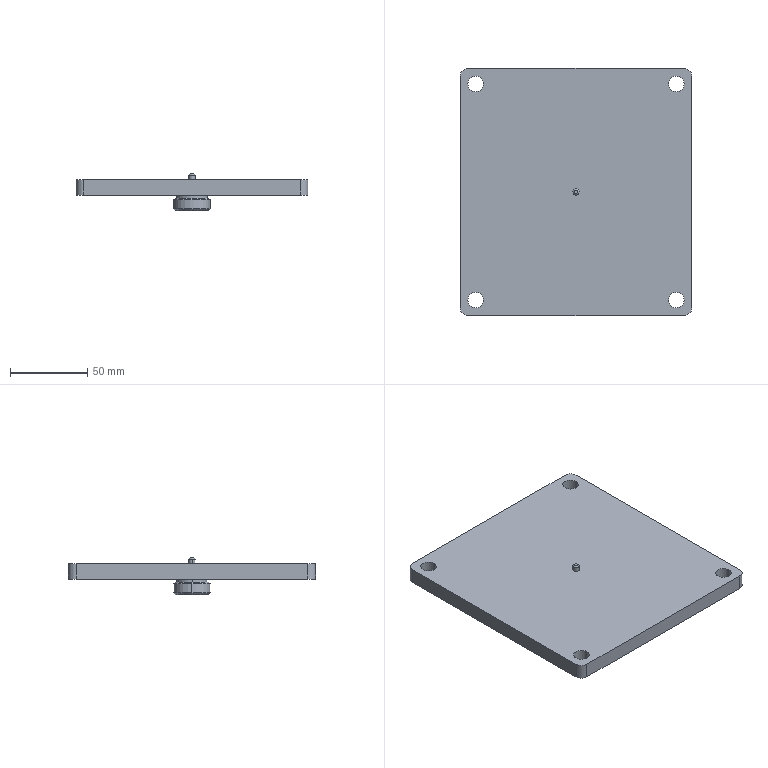Component | SolidWorks | GearboxTopCover-1 | 1 solid | 33 faces | box 150 x 160 x 24 mm | volume 240863 mm3 | cylinder 18 | plane 9 | cone 6 | commonest cylinder face diameters 10 x12 24 x2 4 x2 20 x2
build123d program:
from build123d import *

# Parameters (mm, degrees)
SKETCH1_4_W         = 160
SKETCH1_4_H         = 150
SKETCH1_4_R         = 10
SKETCH1_4_R_2       = 5
BOSS_EXTRUDE1_DEPTH = 10
FILLET1_R           = 5
SKETCH1_3_R         = 10
SKETCH1_3_R_2       = 2
BOSS_EXTRUDE2_DEPTH = 12
SKETCH1_4_2_R       = 2
BOSS_EXTRUDE3_DEPTH = 4
CHAMFER1_SIZE       = 1
SKETCH4_R           = 12
BOSS_EXTRUDE4_DEPTH = 8
CHAMFER2_SIZE       = 1


with BuildPart() as part:
    # Sketch1_4 → Boss-Extrude1 (new body)
    with BuildSketch(Plane(origin=(0, 0, 0), x_dir=(1, 0, 0), z_dir=(0, 1, 0))):
        Rectangle(SKETCH1_4_W, SKETCH1_4_H)
        with Locations(Location((0, 0, 0), (0, 0, 270))):
            Circle(SKETCH1_4_R, mode=Mode.SUBTRACT)
        with Locations(Location((-70, -65, 0), (0, 0, 270))):
            Circle(SKETCH1_4_R_2, mode=Mode.SUBTRACT)
        with Locations(Location((-70, 65, 0), (0, 0, 270))):
            Circle(SKETCH1_4_R_2, mode=Mode.SUBTRACT)
        with Locations(Location((70, -65, 0), (0, 0, 270))):
            Circle(SKETCH1_4_R_2, mode=Mode.SUBTRACT)
        with Locations(Location((70, 65, 0), (0, 0, 270))):
            Circle(SKETCH1_4_R_2, mode=Mode.SUBTRACT)
    extrude(amount=BOSS_EXTRUDE1_DEPTH)

    # Fillet1
    fillet1_edges = [part.edges().sort_by_distance(p)[0] for p in [
        (-80, 5, 75),
        (-80, 5, -75),
        (80, 5, -75),
        (80, 5, 75),
    ]]
    fillet(fillet1_edges, radius=FILLET1_R)

    # Sketch1_3 → Boss-Extrude2 (add)
    # profile 1 of 2: a face of its own
    with BuildSketch(Plane(origin=(0, 0, 0), x_dir=(1, 0, 0), z_dir=(0, 1, 0))):
        with Locations(Location((0, 0, 0), (0, 0, 270))):
            Circle(SKETCH1_3_R)
        Circle(SKETCH1_3_R_2, mode=Mode.SUBTRACT)
    # profile 2 of 2: a face of its own
    with BuildSketch(Plane(origin=(0, 0, 0), x_dir=(1, 0, 0), z_dir=(0, 1, 0))):
        Circle(SKETCH1_3_R_2)
    extrude(amount=BOSS_EXTRUDE2_DEPTH)

    # Sketch1_4 2 → Boss-Extrude3 (add)
    with BuildSketch(Plane(origin=(0, 0, 0), x_dir=(1, 0, 0), z_dir=(0, 1, 0))):
        with Locations(Location((0, 0, 0), (0, 0, 270))):
            Circle(SKETCH1_4_2_R)
    extrude(amount=-BOSS_EXTRUDE3_DEPTH)

    # Chamfer1
    chamfer1_edges = [part.edges().sort_by_distance(p)[0] for p in [
        (0, -4, -2),
    ]]
    chamfer(chamfer1_edges, length=CHAMFER1_SIZE)

    # Sketch4 → Boss-Extrude4 (add)
    with BuildSketch(Plane(origin=(0, 12, 0), x_dir=(1, 0, 0), z_dir=(0, 1, 0))):
        with Locations(Location((0, 0, 0), (0, 0, 270))):
            Circle(SKETCH4_R)
    extrude(amount=BOSS_EXTRUDE4_DEPTH)

    # Chamfer2
    chamfer2_edges = [part.edges().sort_by_distance(p)[0] for p in [
        (0, 12, -12),
        (0, 20, -12),
    ]]
    chamfer(chamfer2_edges, length=CHAMFER2_SIZE)


solid = part.part

# Placed as in the assembly
solid = solid.moved(Location((-40.429, -8.561, -295), (-90, 90, 0)))
STEP:
#1=CARTESIAN_POINT('',(-1.159,-0.3371,-12.402));
#2=VERTEX_POINT('',#1);
#3=CARTESIAN_POINT('',(-2.025,-0.3371,-12.402));
#4=VERTEX_POINT('',#3);
#5=CARTESIAN_POINT('',(-1.592,-0.3371,-12.402));
#6=DIRECTION('',(0.,0.,-1.));
#7=DIRECTION('',(1.,0.,0.));
#8=AXIS2_PLACEMENT_3D('',#5,#6,#7);
#9=CIRCLE('',#8,0.4331);
#10=EDGE_CURVE('',#2,#4,#9,.T.);
#11=ORIENTED_EDGE('',*,*,#10,.F.);
#12=CARTESIAN_POINT('',(-1.119,-0.3371,-12.362));
#13=VERTEX_POINT('',#12);
#14=CARTESIAN_POINT('',(-1.159,-0.3371,-12.402));
#15=DIRECTION('',(0.7071,-0.,0.7071));
#16=VECTOR('',#15,39.37);
#17=LINE('',#14,#16);
#18=EDGE_CURVE('',#2,#13,#17,.T.);
#19=ORIENTED_EDGE('',*,*,#18,.T.);
#20=CARTESIAN_POINT('',(-2.064,-0.3371,-12.362));
#21=VERTEX_POINT('',#20);
#22=CARTESIAN_POINT('',(-1.592,-0.3371,-12.362));
#23=DIRECTION('',(-0.,-0.,1.));
#24=DIRECTION('',(1.,0.,0.));
#25=AXIS2_PLACEMENT_3D('',#22,#23,#24);
#26=CIRCLE('',#25,0.4724);
#27=EDGE_CURVE('',#21,#13,#26,.T.);
#28=ORIENTED_EDGE('',*,*,#27,.F.);
#29=CARTESIAN_POINT('',(-2.025,-0.3371,-12.402));
#30=DIRECTION('',(-0.7071,-0.,0.7071));
#31=VECTOR('',#30,39.37);
#32=LINE('',#29,#31);
#33=EDGE_CURVE('',#4,#21,#32,.T.);
#34=ORIENTED_EDGE('',*,*,#33,.F.);
#35=EDGE_LOOP('',(#11,#19,#28,#34));
#36=FACE_OUTER_BOUND('',#35,.T.);
#37=CARTESIAN_POINT('',(-1.592,-0.3371,-12.402));
#38=DIRECTION('',(-0.,-0.,1.));
#39=DIRECTION('',(-1.,0.,0.));
#40=AXIS2_PLACEMENT_3D('',#37,#38,#39);
#41=CONICAL_SURFACE('',#40,0.4331,0.7854);
#42=ADVANCED_FACE('',(#36),#41,.T.);
#43=CARTESIAN_POINT('',(-2.025,-0.3371,-12.087));
#44=VERTEX_POINT('',#43);
#45=CARTESIAN_POINT('',(-1.159,-0.3371,-12.087));
#46=VERTEX_POINT('',#45);
#47=CARTESIAN_POINT('',(-1.592,-0.3371,-12.087));
#48=DIRECTION('',(-0.,-0.,1.));
#49=DIRECTION('',(1.,0.,0.));
#50=AXIS2_PLACEMENT_3D('',#47,#48,#49);
#51=CIRCLE('',#50,0.4331);
#52=EDGE_CURVE('',#44,#46,#51,.T.);
#53=ORIENTED_EDGE('',*,*,#52,.F.);
#54=CARTESIAN_POINT('',(-2.064,-0.3371,-12.126));
#55=VERTEX_POINT('',#54);
#56=CARTESIAN_POINT('',(-2.064,-0.3371,-12.126));
#57=DIRECTION('',(-0.7071,-0.,-0.7071));
#58=VECTOR('',#57,39.37);
#59=LINE('',#56,#58);
#60=EDGE_CURVE('',#44,#55,#59,.T.);
#61=ORIENTED_EDGE('',*,*,#60,.T.);
#62=CARTESIAN_POINT('',(-1.119,-0.3371,-12.126));
#63=VERTEX_POINT('',#62);
#64=CARTESIAN_POINT('',(-1.592,-0.3371,-12.126));
#65=DIRECTION('',(0.,0.,-1.));
#66=DIRECTION('',(1.,0.,0.));
#67=AXIS2_PLACEMENT_3D('',#64,#65,#66);
#68=CIRCLE('',#67,0.4724);
#69=EDGE_CURVE('',#63,#55,#68,.T.);
#70=ORIENTED_EDGE('',*,*,#69,.F.);
#71=CARTESIAN_POINT('',(-1.119,-0.3371,-12.126));
#72=DIRECTION('',(0.7071,0.,-0.7071));
#73=VECTOR('',#72,39.37);
#74=LINE('',#71,#73);
#75=EDGE_CURVE('',#46,#63,#74,.T.);
#76=ORIENTED_EDGE('',*,*,#75,.F.);
#77=EDGE_LOOP('',(#53,#61,#70,#76));
#78=FACE_OUTER_BOUND('',#77,.T.);
#79=CARTESIAN_POINT('',(-1.592,-0.3371,-12.126));
#80=DIRECTION('',(0.,0.,-1.));
#81=DIRECTION('',(1.,0.,0.));
#82=AXIS2_PLACEMENT_3D('',#79,#80,#81);
#83=CONICAL_SURFACE('',#82,0.4724,0.7854);
#84=ADVANCED_FACE('',(#78),#83,.T.);
#85=ORIENTED_EDGE('',*,*,#27,.T.);
#86=CARTESIAN_POINT('',(-1.119,-0.3371,-12.402));
#87=DIRECTION('',(-0.,-0.,1.));
#88=VECTOR('',#87,39.37);
#89=LINE('',#86,#88);
#90=EDGE_CURVE('',#13,#63,#89,.T.);
#91=ORIENTED_EDGE('',*,*,#90,.T.);
#92=ORIENTED_EDGE('',*,*,#69,.T.);
#93=CARTESIAN_POINT('',(-2.064,-0.3371,-12.402));
#94=DIRECTION('',(-0.,-0.,1.));
#95=VECTOR('',#94,39.37);
#96=LINE('',#93,#95);
#97=EDGE_CURVE('',#21,#55,#96,.T.);
#98=ORIENTED_EDGE('',*,*,#97,.F.);
#99=EDGE_LOOP('',(#85,#91,#92,#98));
#100=FACE_OUTER_BOUND('',#99,.T.);
#101=CARTESIAN_POINT('',(-1.592,-0.3371,-12.402));
#102=DIRECTION('',(-0.,-0.,1.));
#103=DIRECTION('',(-1.,0.,0.));
#104=AXIS2_PLACEMENT_3D('',#101,#102,#103);
#105=CYLINDRICAL_SURFACE('',#104,0.4724);
#106=ADVANCED_FACE('',(#100),#105,.T.);
#107=CARTESIAN_POINT('',(-1.631,-0.3371,-11.457));
#108=VERTEX_POINT('',#107);
#109=CARTESIAN_POINT('',(-1.552,-0.3371,-11.457));
#110=VERTEX_POINT('',#109);
#111=CARTESIAN_POINT('',(-1.592,-0.3371,-11.457));
#112=DIRECTION('',(-0.,-0.,1.));
#113=DIRECTION('',(1.,0.,0.));
#114=AXIS2_PLACEMENT_3D('',#111,#112,#113);
#115=CIRCLE('',#114,0.03937);
#116=EDGE_CURVE('',#108,#110,#115,.T.);
#117=ORIENTED_EDGE('',*,*,#116,.F.);
#118=CARTESIAN_POINT('',(-1.67,-0.3371,-11.496));
#119=VERTEX_POINT('',#118);
#120=CARTESIAN_POINT('',(-1.67,-0.3371,-11.496));
#121=DIRECTION('',(-0.7071,-0.,-0.7071));
#122=VECTOR('',#121,39.37);
#123=LINE('',#120,#122);
#124=EDGE_CURVE('',#108,#119,#123,.T.);
#125=ORIENTED_EDGE('',*,*,#124,.T.);
#126=CARTESIAN_POINT('',(-1.513,-0.3371,-11.496));
#127=VERTEX_POINT('',#126);
#128=CARTESIAN_POINT('',(-1.592,-0.3371,-11.496));
#129=DIRECTION('',(0.,0.,-1.));
#130=DIRECTION('',(1.,0.,0.));
#131=AXIS2_PLACEMENT_3D('',#128,#129,#130);
#132=CIRCLE('',#131,0.07874);
#133=EDGE_CURVE('',#127,#119,#132,.T.);
#134=ORIENTED_EDGE('',*,*,#133,.F.);
#135=CARTESIAN_POINT('',(-1.513,-0.3371,-11.496));
#136=DIRECTION('',(0.7071,0.,-0.7071));
#137=VECTOR('',#136,39.37);
#138=LINE('',#135,#137);
#139=EDGE_CURVE('',#110,#127,#138,.T.);
#140=ORIENTED_EDGE('',*,*,#139,.F.);
#141=EDGE_LOOP('',(#117,#125,#134,#140));
#142=FACE_OUTER_BOUND('',#141,.T.);
#143=CARTESIAN_POINT('',(-1.592,-0.3371,-11.496));
#144=DIRECTION('',(0.,0.,-1.));
#145=DIRECTION('',(1.,0.,0.));
#146=AXIS2_PLACEMENT_3D('',#143,#144,#145);
#147=CONICAL_SURFACE('',#146,0.07874,0.7854);
#148=ADVANCED_FACE('',(#142),#147,.T.);
#149=ORIENTED_EDGE('',*,*,#133,.T.);
#150=CARTESIAN_POINT('',(-1.67,-0.3371,-11.614));
#151=VERTEX_POINT('',#150);
#152=CARTESIAN_POINT('',(-1.67,-0.3371,-11.457));
#153=DIRECTION('',(0.,0.,-1.));
#154=VECTOR('',#153,39.37);
#155=LINE('',#152,#154);
#156=EDGE_CURVE('',#119,#151,#155,.T.);
#157=ORIENTED_EDGE('',*,*,#156,.T.);
#158=CARTESIAN_POINT('',(-1.513,-0.3371,-11.614));
#159=VERTEX_POINT('',#158);
#160=CARTESIAN_POINT('',(-1.592,-0.3371,-11.614));
#161=DIRECTION('',(0.,0.,-1.));
#162=DIRECTION('',(1.,0.,0.));
#163=AXIS2_PLACEMENT_3D('',#160,#161,#162);
#164=CIRCLE('',#163,0.07874);
#165=EDGE_CURVE('',#159,#151,#164,.T.);
#166=ORIENTED_EDGE('',*,*,#165,.F.);
#167=CARTESIAN_POINT('',(-1.513,-0.3371,-11.457));
#168=DIRECTION('',(0.,0.,-1.));
#169=VECTOR('',#168,39.37);
#170=LINE('',#167,#169);
#171=EDGE_CURVE('',#127,#159,#170,.T.);
#172=ORIENTED_EDGE('',*,*,#171,.F.);
#173=EDGE_LOOP('',(#149,#157,#166,#172));
#174=FACE_OUTER_BOUND('',#173,.T.);
#175=CARTESIAN_POINT('',(-1.592,-0.3371,-11.457));
#176=DIRECTION('',(0.,0.,-1.));
#177=DIRECTION('',(1.,0.,0.));
#178=AXIS2_PLACEMENT_3D('',#175,#176,#177);
#179=CYLINDRICAL_SURFACE('',#178,0.07874);
#180=ADVANCED_FACE('',(#174),#179,.T.);
#181=CARTESIAN_POINT('',(-1.198,-0.3371,-12.087));
#182=VERTEX_POINT('',#181);
#183=CARTESIAN_POINT('',(-1.985,-0.3371,-12.087));
#184=VERTEX_POINT('',#183);
#185=CARTESIAN_POINT('',(-1.592,-0.3371,-12.087));
#186=DIRECTION('',(0.,0.,-1.));
#187=DIRECTION('',(1.,0.,0.));
#188=AXIS2_PLACEMENT_3D('',#185,#186,#187);
#189=CIRCLE('',#188,0.3937);
#190=EDGE_CURVE('',#182,#184,#189,.T.);
#191=ORIENTED_EDGE('',*,*,#190,.F.);
#192=CARTESIAN_POINT('',(-1.198,-0.3371,-12.008));
#193=VERTEX_POINT('',#192);
#194=CARTESIAN_POINT('',(-1.198,-0.3371,-12.087));
#195=DIRECTION('',(-0.,-0.,1.));
#196=VECTOR('',#195,39.37);
#197=LINE('',#194,#196);
#198=EDGE_CURVE('',#182,#193,#197,.T.);
#199=ORIENTED_EDGE('',*,*,#198,.T.);
#200=CARTESIAN_POINT('',(-1.985,-0.3371,-12.008));
#201=VERTEX_POINT('',#200);
#202=CARTESIAN_POINT('',(-1.592,-0.3371,-12.008));
#203=DIRECTION('',(0.,0.,-1.));
#204=DIRECTION('',(1.,0.,0.));
#205=AXIS2_PLACEMENT_3D('',#202,#203,#204);
#206=CIRCLE('',#205,0.3937);
#207=EDGE_CURVE('',#193,#201,#206,.T.);
#208=ORIENTED_EDGE('',*,*,#207,.T.);
#209=CARTESIAN_POINT('',(-1.985,-0.3371,-12.087));
#210=DIRECTION('',(-0.,-0.,1.));
#211=VECTOR('',#210,39.37);
#212=LINE('',#209,#211);
#213=EDGE_CURVE('',#184,#201,#212,.T.);
#214=ORIENTED_EDGE('',*,*,#213,.F.);
#215=EDGE_LOOP('',(#191,#199,#208,#214));
#216=FACE_OUTER_BOUND('',#215,.T.);
#217=CARTESIAN_POINT('',(-1.592,-0.3371,-12.087));
#218=DIRECTION('',(-0.,-0.,1.));
#219=DIRECTION('',(-1.,0.,0.));
#220=AXIS2_PLACEMENT_3D('',#217,#218,#219);
#221=CYLINDRICAL_SURFACE('',#220,0.3937);
#222=ADVANCED_FACE('',(#216),#221,.T.);
#223=CARTESIAN_POINT('',(-3.954,-3.093,-12.008));
#224=VERTEX_POINT('',#223);
#225=CARTESIAN_POINT('',(-4.348,-3.093,-12.008));
#226=VERTEX_POINT('',#225);
#227=CARTESIAN_POINT('',(-4.151,-3.093,-12.008));
#228=DIRECTION('',(-0.,-0.,1.));
#229=DIRECTION('',(1.,0.,0.));
#230=AXIS2_PLACEMENT_3D('',#227,#228,#229);
#231=CIRCLE('',#230,0.1969);
#232=EDGE_CURVE('',#224,#226,#231,.T.);
#233=ORIENTED_EDGE('',*,*,#232,.F.);
#234=CARTESIAN_POINT('',(-3.954,-3.093,-11.614));
#235=VERTEX_POINT('',#234);
#236=CARTESIAN_POINT('',(-3.954,-3.093,-12.008));
#237=DIRECTION('',(-0.,-0.,1.));
#238=VECTOR('',#237,39.37);
#239=LINE('',#236,#238);
#240=EDGE_CURVE('',#224,#235,#239,.T.);
#241=ORIENTED_EDGE('',*,*,#240,.T.);
#242=CARTESIAN_POINT('',(-4.348,-3.093,-11.614));
#243=VERTEX_POINT('',#242);
#244=CARTESIAN_POINT('',(-4.151,-3.093,-11.614));
#245=DIRECTION('',(-0.,-0.,1.));
#246=DIRECTION('',(1.,0.,0.));
#247=AXIS2_PLACEMENT_3D('',#244,#245,#246);
#248=CIRCLE('',#247,0.1969);
#249=EDGE_CURVE('',#235,#243,#248,.T.);
#250=ORIENTED_EDGE('',*,*,#249,.T.);
#251=CARTESIAN_POINT('',(-4.348,-3.093,-12.008));
#252=DIRECTION('',(-0.,-0.,1.));
#253=VECTOR('',#252,39.37);
#254=LINE('',#251,#253);
#255=EDGE_CURVE('',#226,#243,#254,.T.);
#256=ORIENTED_EDGE('',*,*,#255,.F.);
#257=EDGE_LOOP('',(#233,#241,#250,#256));
#258=FACE_OUTER_BOUND('',#257,.T.);
#259=CARTESIAN_POINT('',(-4.151,-3.093,-12.008));
#260=DIRECTION('',(-0.,-0.,1.));
#261=DIRECTION('',(-1.,0.,0.));
#262=AXIS2_PLACEMENT_3D('',#259,#260,#261);
#263=CYLINDRICAL_SURFACE('',#262,0.1969);
#264=ADVANCED_FACE('',(#258),#263,.F.);
#265=CARTESIAN_POINT('',(1.164,2.419,-12.008));
#266=VERTEX_POINT('',#265);
#267=CARTESIAN_POINT('',(0.7705,2.419,-12.008));
#268=VERTEX_POINT('',#267);
#269=CARTESIAN_POINT('',(0.9674,2.419,-12.008));
#270=DIRECTION('',(-0.,-0.,1.));
#271=DIRECTION('',(1.,0.,0.));
#272=AXIS2_PLACEMENT_3D('',#269,#270,#271);
#273=CIRCLE('',#272,0.1969);
#274=EDGE_CURVE('',#266,#268,#273,.T.);
#275=ORIENTED_EDGE('',*,*,#274,.F.);
#276=CARTESIAN_POINT('',(1.164,2.419,-11.614));
#277=VERTEX_POINT('',#276);
#278=CARTESIAN_POINT('',(1.164,2.419,-12.008));
#279=DIRECTION('',(-0.,-0.,1.));
#280=VECTOR('',#279,39.37);
#281=LINE('',#278,#280);
#282=EDGE_CURVE('',#266,#277,#281,.T.);
#283=ORIENTED_EDGE('',*,*,#282,.T.);
#284=CARTESIAN_POINT('',(0.7705,2.419,-11.614));
#285=VERTEX_POINT('',#284);
#286=CARTESIAN_POINT('',(0.9674,2.419,-11.614));
#287=DIRECTION('',(-0.,-0.,1.));
#288=DIRECTION('',(1.,0.,0.));
#289=AXIS2_PLACEMENT_3D('',#286,#287,#288);
#290=CIRCLE('',#289,0.1969);
#291=EDGE_CURVE('',#277,#285,#290,.T.);
#292=ORIENTED_EDGE('',*,*,#291,.T.);
#293=CARTESIAN_POINT('',(0.7705,2.419,-12.008));
#294=DIRECTION('',(-0.,-0.,1.));
#295=VECTOR('',#294,39.37);
#296=LINE('',#293,#295);
#297=EDGE_CURVE('',#268,#285,#296,.T.);
#298=ORIENTED_EDGE('',*,*,#297,.F.);
#299=EDGE_LOOP('',(#275,#283,#292,#298));
#300=FACE_OUTER_BOUND('',#299,.T.);
#301=CARTESIAN_POINT('',(0.9674,2.419,-12.008));
#302=DIRECTION('',(-0.,-0.,1.));
#303=DIRECTION('',(-1.,0.,0.));
#304=AXIS2_PLACEMENT_3D('',#301,#302,#303);
#305=CYLINDRICAL_SURFACE('',#304,0.1969);
#306=ADVANCED_FACE('',(#300),#305,.F.);
#307=CARTESIAN_POINT('',(-4.348,2.419,-12.008));
#308=VERTEX_POINT('',#307);
#309=CARTESIAN_POINT('',(-3.954,2.419,-12.008));
#310=VERTEX_POINT('',#309);
#311=CARTESIAN_POINT('',(-4.151,2.419,-12.008));
#312=DIRECTION('',(0.,0.,-1.));
#313=DIRECTION('',(1.,0.,0.));
#314=AXIS2_PLACEMENT_3D('',#311,#312,#313);
#315=CIRCLE('',#314,0.1969);
#316=EDGE_CURVE('',#308,#310,#315,.T.);
#317=ORIENTED_EDGE('',*,*,#316,.T.);
#318=CARTESIAN_POINT('',(-3.954,2.419,-11.614));
#319=VERTEX_POINT('',#318);
#320=CARTESIAN_POINT('',(-3.954,2.419,-12.008));
#321=DIRECTION('',(-0.,-0.,1.));
#322=VECTOR('',#321,39.37);
#323=LINE('',#320,#322);
#324=EDGE_CURVE('',#310,#319,#323,.T.);
#325=ORIENTED_EDGE('',*,*,#324,.T.);
#326=CARTESIAN_POINT('',(-4.348,2.419,-11.614));
#327=VERTEX_POINT('',#326);
#328=CARTESIAN_POINT('',(-4.151,2.419,-11.614));
#329=DIRECTION('',(0.,0.,-1.));
#330=DIRECTION('',(1.,0.,0.));
#331=AXIS2_PLACEMENT_3D('',#328,#329,#330);
#332=CIRCLE('',#331,0.1969);
#333=EDGE_CURVE('',#327,#319,#332,.T.);
#334=ORIENTED_EDGE('',*,*,#333,.F.);
#335=CARTESIAN_POINT('',(-4.348,2.419,-12.008));
#336=DIRECTION('',(-0.,-0.,1.));
#337=VECTOR('',#336,39.37);
#338=LINE('',#335,#337);
#339=EDGE_CURVE('',#308,#327,#338,.T.);
#340=ORIENTED_EDGE('',*,*,#339,.F.);
#341=EDGE_LOOP('',(#317,#325,#334,#340));
#342=FACE_OUTER_BOUND('',#341,.T.);
#343=CARTESIAN_POINT('',(-4.151,2.419,-12.008));
#344=DIRECTION('',(-0.,-0.,1.));
#345=DIRECTION('',(-1.,0.,0.));
#346=AXIS2_PLACEMENT_3D('',#343,#344,#345);
#347=CYLINDRICAL_SURFACE('',#346,0.1969);
#348=ADVANCED_FACE('',(#342),#347,.F.);
#349=CARTESIAN_POINT('',(0.7705,-3.093,-12.008));
#350=VERTEX_POINT('',#349);
#351=CARTESIAN_POINT('',(1.164,-3.093,-12.008));
#352=VERTEX_POINT('',#351);
#353=CARTESIAN_POINT('',(0.9674,-3.093,-12.008));
#354=DIRECTION('',(0.,0.,-1.));
#355=DIRECTION('',(1.,0.,0.));
#356=AXIS2_PLACEMENT_3D('',#353,#354,#355);
#357=CIRCLE('',#356,0.1969);
#358=EDGE_CURVE('',#350,#352,#357,.T.);
#359=ORIENTED_EDGE('',*,*,#358,.T.);
#360=CARTESIAN_POINT('',(1.164,-3.093,-11.614));
#361=VERTEX_POINT('',#360);
#362=CARTESIAN_POINT('',(1.164,-3.093,-12.008));
#363=DIRECTION('',(-0.,-0.,1.));
#364=VECTOR('',#363,39.37);
#365=LINE('',#362,#364);
#366=EDGE_CURVE('',#352,#361,#365,.T.);
#367=ORIENTED_EDGE('',*,*,#366,.T.);
#368=CARTESIAN_POINT('',(0.7705,-3.093,-11.614));
#369=VERTEX_POINT('',#368);
#370=CARTESIAN_POINT('',(0.9674,-3.093,-11.614));
#371=DIRECTION('',(0.,0.,-1.));
#372=DIRECTION('',(1.,0.,0.));
#373=AXIS2_PLACEMENT_3D('',#370,#371,#372);
#374=CIRCLE('',#373,0.1969);
#375=EDGE_CURVE('',#369,#361,#374,.T.);
#376=ORIENTED_EDGE('',*,*,#375,.F.);
#377=CARTESIAN_POINT('',(0.7705,-3.093,-12.008));
#378=DIRECTION('',(-0.,-0.,1.));
#379=VECTOR('',#378,39.37);
#380=LINE('',#377,#379);
#381=EDGE_CURVE('',#350,#369,#380,.T.);
#382=ORIENTED_EDGE('',*,*,#381,.F.);
#383=EDGE_LOOP('',(#359,#367,#376,#382));
#384=FACE_OUTER_BOUND('',#383,.T.);
#385=CARTESIAN_POINT('',(0.9674,-3.093,-12.008));
#386=DIRECTION('',(-0.,-0.,1.));
#387=DIRECTION('',(-1.,0.,0.));
#388=AXIS2_PLACEMENT_3D('',#385,#386,#387);
#389=CYLINDRICAL_SURFACE('',#388,0.1969);
#390=ADVANCED_FACE('',(#384),#389,.F.);
#391=CARTESIAN_POINT('',(1.361,2.616,-12.008));
#392=VERTEX_POINT('',#391);
#393=CARTESIAN_POINT('',(1.361,-3.29,-12.008));
#394=VERTEX_POINT('',#393);
#395=CARTESIAN_POINT('',(1.361,-0.3371,-12.008));
#396=DIRECTION('',(0.,-1.,0.));
#397=VECTOR('',#396,39.37);
#398=LINE('',#395,#397);
#399=EDGE_CURVE('',#392,#394,#398,.T.);
#400=ORIENTED_EDGE('',*,*,#399,.F.);
#401=CARTESIAN_POINT('',(1.361,2.616,-11.614));
#402=VERTEX_POINT('',#401);
#403=CARTESIAN_POINT('',(1.361,2.616,-11.614));
#404=DIRECTION('',(-0.,-0.,1.));
#405=VECTOR('',#404,39.37);
#406=LINE('',#403,#405);
#407=EDGE_CURVE('',#392,#402,#406,.T.);
#408=ORIENTED_EDGE('',*,*,#407,.T.);
#409=CARTESIAN_POINT('',(1.361,-3.29,-11.614));
#410=VERTEX_POINT('',#409);
#411=CARTESIAN_POINT('',(1.361,-0.3371,-11.614));
#412=DIRECTION('',(0.,-1.,0.));
#413=VECTOR('',#412,39.37);
#414=LINE('',#411,#413);
#415=EDGE_CURVE('',#402,#410,#414,.T.);
#416=ORIENTED_EDGE('',*,*,#415,.T.);
#417=CARTESIAN_POINT('',(1.361,-3.29,-12.008));
#418=DIRECTION('',(0.,0.,-1.));
#419=VECTOR('',#418,39.37);
#420=LINE('',#417,#419);
#421=EDGE_CURVE('',#410,#394,#420,.T.);
#422=ORIENTED_EDGE('',*,*,#421,.T.);
#423=EDGE_LOOP('',(#400,#408,#416,#422));
#424=FACE_OUTER_BOUND('',#423,.T.);
#425=CARTESIAN_POINT('',(1.361,-0.3371,-12.008));
#426=DIRECTION('',(-1.,-0.,-0.));
#427=DIRECTION('',(-0.,1.,0.));
#428=AXIS2_PLACEMENT_3D('',#425,#426,#427);
#429=PLANE('',#428);
#430=ADVANCED_FACE('',(#424),#429,.F.);
#431=CARTESIAN_POINT('',(1.164,-3.487,-11.614));
#432=VERTEX_POINT('',#431);
#433=CARTESIAN_POINT('',(-4.348,-3.487,-11.614));
#434=VERTEX_POINT('',#433);
#435=CARTESIAN_POINT('',(-1.592,-3.487,-11.614));
#436=DIRECTION('',(-1.,-0.,-0.));
#437=VECTOR('',#436,39.37);
#438=LINE('',#435,#437);
#439=EDGE_CURVE('',#432,#434,#438,.T.);
#440=ORIENTED_EDGE('',*,*,#439,.T.);
#441=CARTESIAN_POINT('',(-4.348,-3.487,-12.008));
#442=VERTEX_POINT('',#441);
#443=CARTESIAN_POINT('',(-4.348,-3.487,-12.008));
#444=DIRECTION('',(0.,0.,-1.));
#445=VECTOR('',#444,39.37);
#446=LINE('',#443,#445);
#447=EDGE_CURVE('',#434,#442,#446,.T.);
#448=ORIENTED_EDGE('',*,*,#447,.T.);
#449=CARTESIAN_POINT('',(1.164,-3.487,-12.008));
#450=VERTEX_POINT('',#449);
#451=CARTESIAN_POINT('',(-1.592,-3.487,-12.008));
#452=DIRECTION('',(-1.,-0.,-0.));
#453=VECTOR('',#452,39.37);
#454=LINE('',#451,#453);
#455=EDGE_CURVE('',#450,#442,#454,.T.);
#456=ORIENTED_EDGE('',*,*,#455,.F.);
#457=CARTESIAN_POINT('',(1.164,-3.487,-12.008));
#458=DIRECTION('',(-0.,-0.,1.));
#459=VECTOR('',#458,39.37);
#460=LINE('',#457,#459);
#461=EDGE_CURVE('',#450,#432,#460,.T.);
#462=ORIENTED_EDGE('',*,*,#461,.T.);
#463=EDGE_LOOP('',(#440,#448,#456,#462));
#464=FACE_OUTER_BOUND('',#463,.T.);
#465=CARTESIAN_POINT('',(-1.592,-3.487,-12.008));
#466=DIRECTION('',(-0.,1.,0.));
#467=DIRECTION('',(1.,0.,0.));
#468=AXIS2_PLACEMENT_3D('',#465,#466,#467);
#469=PLANE('',#468);
#470=ADVANCED_FACE('',(#464),#469,.F.);
#471=CARTESIAN_POINT('',(-4.544,2.616,-11.614));
#472=VERTEX_POINT('',#471);
#473=CARTESIAN_POINT('',(-4.544,-3.29,-11.614));
#474=VERTEX_POINT('',#473);
#475=CARTESIAN_POINT('',(-4.544,-0.3371,-11.614));
#476=DIRECTION('',(0.,-1.,0.));
#477=VECTOR('',#476,39.37);
#478=LINE('',#475,#477);
#479=EDGE_CURVE('',#472,#474,#478,.T.);
#480=ORIENTED_EDGE('',*,*,#479,.F.);
#481=CARTESIAN_POINT('',(-4.544,2.616,-12.008));
#482=VERTEX_POINT('',#481);
#483=CARTESIAN_POINT('',(-4.544,2.616,-12.008));
#484=DIRECTION('',(0.,0.,-1.));
#485=VECTOR('',#484,39.37);
#486=LINE('',#483,#485);
#487=EDGE_CURVE('',#472,#482,#486,.T.);
#488=ORIENTED_EDGE('',*,*,#487,.T.);
#489=CARTESIAN_POINT('',(-4.544,-3.29,-12.008));
#490=VERTEX_POINT('',#489);
#491=CARTESIAN_POINT('',(-4.544,-0.3371,-12.008));
#492=DIRECTION('',(0.,-1.,0.));
#493=VECTOR('',#492,39.37);
#494=LINE('',#491,#493);
#495=EDGE_CURVE('',#482,#490,#494,.T.);
#496=ORIENTED_EDGE('',*,*,#495,.T.);
#497=CARTESIAN_POINT('',(-4.544,-3.29,-11.614));
#498=DIRECTION('',(-0.,-0.,1.));
#499=VECTOR('',#498,39.37);
#500=LINE('',#497,#499);
#501=EDGE_CURVE('',#490,#474,#500,.T.);
#502=ORIENTED_EDGE('',*,*,#501,.T.);
#503=EDGE_LOOP('',(#480,#488,#496,#502));
#504=FACE_OUTER_BOUND('',#503,.T.);
#505=CARTESIAN_POINT('',(-4.544,-0.3371,-12.008));
#506=DIRECTION('',(-1.,-0.,-0.));
#507=DIRECTION('',(-0.,1.,0.));
#508=AXIS2_PLACEMENT_3D('',#505,#506,#507);
#509=PLANE('',#508);
#510=ADVANCED_FACE('',(#504),#509,.T.);
#511=ORIENTED_EDGE('',*,*,#366,.F.);
#512=CARTESIAN_POINT('',(0.9674,-3.093,-12.008));
#513=DIRECTION('',(0.,0.,-1.));
#514=DIRECTION('',(1.,0.,0.));
#515=AXIS2_PLACEMENT_3D('',#512,#513,#514);
#516=CIRCLE('',#515,0.1969);
#517=EDGE_CURVE('',#352,#350,#516,.T.);
#518=ORIENTED_EDGE('',*,*,#517,.T.);
#519=ORIENTED_EDGE('',*,*,#381,.T.);
#520=CARTESIAN_POINT('',(0.9674,-3.093,-11.614));
#521=DIRECTION('',(0.,0.,-1.));
#522=DIRECTION('',(1.,0.,0.));
#523=AXIS2_PLACEMENT_3D('',#520,#521,#522);
#524=CIRCLE('',#523,0.1969);
#525=EDGE_CURVE('',#361,#369,#524,.T.);
#526=ORIENTED_EDGE('',*,*,#525,.F.);
#527=EDGE_LOOP('',(#511,#518,#519,#526));
#528=FACE_OUTER_BOUND('',#527,.T.);
#529=CARTESIAN_POINT('',(0.9674,-3.093,-12.008));
#530=DIRECTION('',(-0.,-0.,1.));
#531=DIRECTION('',(-1.,0.,0.));
#532=AXIS2_PLACEMENT_3D('',#529,#530,#531);
#533=CYLINDRICAL_SURFACE('',#532,0.1969);
#534=ADVANCED_FACE('',(#528),#533,.F.);
#535=CARTESIAN_POINT('',(1.164,2.813,-11.614));
#536=VERTEX_POINT('',#535);
#537=CARTESIAN_POINT('',(-4.348,2.813,-11.614));
#538=VERTEX_POINT('',#537);
#539=CARTESIAN_POINT('',(-1.592,2.813,-11.614));
#540=DIRECTION('',(-1.,-0.,-0.));
#541=VECTOR('',#540,39.37);
#542=LINE('',#539,#541);
#543=EDGE_CURVE('',#536,#538,#542,.T.);
#544=ORIENTED_EDGE('',*,*,#543,.F.);
#545=CARTESIAN_POINT('',(1.164,2.813,-12.008));
#546=VERTEX_POINT('',#545);
#547=CARTESIAN_POINT('',(1.164,2.813,-12.008));
#548=DIRECTION('',(0.,0.,-1.));
#549=VECTOR('',#548,39.37);
#550=LINE('',#547,#549);
#551=EDGE_CURVE('',#536,#546,#550,.T.);
#552=ORIENTED_EDGE('',*,*,#551,.T.);
#553=CARTESIAN_POINT('',(-4.348,2.813,-12.008));
#554=VERTEX_POINT('',#553);
#555=CARTESIAN_POINT('',(-1.592,2.813,-12.008));
#556=DIRECTION('',(-1.,-0.,-0.));
#557=VECTOR('',#556,39.37);
#558=LINE('',#555,#557);
#559=EDGE_CURVE('',#546,#554,#558,.T.);
#560=ORIENTED_EDGE('',*,*,#559,.T.);
#561=CARTESIAN_POINT('',(-4.348,2.813,-12.008));
#562=DIRECTION('',(-0.,-0.,1.));
#563=VECTOR('',#562,39.37);
#564=LINE('',#561,#563);
#565=EDGE_CURVE('',#554,#538,#564,.T.);
#566=ORIENTED_EDGE('',*,*,#565,.T.);
#567=EDGE_LOOP('',(#544,#552,#560,#566));
#568=FACE_OUTER_BOUND('',#567,.T.);
#569=CARTESIAN_POINT('',(-1.592,2.813,-12.008));
#570=DIRECTION('',(-0.,1.,0.));
#571=DIRECTION('',(1.,0.,0.));
#572=AXIS2_PLACEMENT_3D('',#569,#570,#571);
#573=PLANE('',#572);
#574=ADVANCED_FACE('',(#568),#573,.T.);
#575=ORIENTED_EDGE('',*,*,#324,.F.);
#576=CARTESIAN_POINT('',(-4.151,2.419,-12.008));
#577=DIRECTION('',(0.,0.,-1.));
#578=DIRECTION('',(1.,0.,0.));
#579=AXIS2_PLACEMENT_3D('',#576,#577,#578);
#580=CIRCLE('',#579,0.1969);
#581=EDGE_CURVE('',#310,#308,#580,.T.);
#582=ORIENTED_EDGE('',*,*,#581,.T.);
#583=ORIENTED_EDGE('',*,*,#339,.T.);
#584=CARTESIAN_POINT('',(-4.151,2.419,-11.614));
#585=DIRECTION('',(0.,0.,-1.));
#586=DIRECTION('',(1.,0.,0.));
#587=AXIS2_PLACEMENT_3D('',#584,#585,#586);
#588=CIRCLE('',#587,0.1969);
#589=EDGE_CURVE('',#319,#327,#588,.T.);
#590=ORIENTED_EDGE('',*,*,#589,.F.);
#591=EDGE_LOOP('',(#575,#582,#583,#590));
#592=FACE_OUTER_BOUND('',#591,.T.);
#593=CARTESIAN_POINT('',(-4.151,2.419,-12.008));
#594=DIRECTION('',(-0.,-0.,1.));
#595=DIRECTION('',(-1.,0.,0.));
#596=AXIS2_PLACEMENT_3D('',#593,#594,#595);
#597=CYLINDRICAL_SURFACE('',#596,0.1969);
#598=ADVANCED_FACE('',(#592),#597,.F.);
#599=ORIENTED_EDGE('',*,*,#282,.F.);
#600=CARTESIAN_POINT('',(0.9674,2.419,-12.008));
#601=DIRECTION('',(-0.,-0.,1.));
#602=DIRECTION('',(1.,0.,0.));
#603=AXIS2_PLACEMENT_3D('',#600,#601,#602);
#604=CIRCLE('',#603,0.1969);
#605=EDGE_CURVE('',#268,#266,#604,.T.);
#606=ORIENTED_EDGE('',*,*,#605,.F.);
#607=ORIENTED_EDGE('',*,*,#297,.T.);
#608=CARTESIAN_POINT('',(0.9674,2.419,-11.614));
#609=DIRECTION('',(-0.,-0.,1.));
#610=DIRECTION('',(1.,0.,0.));
#611=AXIS2_PLACEMENT_3D('',#608,#609,#610);
#612=CIRCLE('',#611,0.1969);
#613=EDGE_CURVE('',#285,#277,#612,.T.);
#614=ORIENTED_EDGE('',*,*,#613,.T.);
#615=EDGE_LOOP('',(#599,#606,#607,#614));
#616=FACE_OUTER_BOUND('',#615,.T.);
#617=CARTESIAN_POINT('',(0.9674,2.419,-12.008));
#618=DIRECTION('',(-0.,-0.,1.));
#619=DIRECTION('',(-1.,0.,0.));
#620=AXIS2_PLACEMENT_3D('',#617,#618,#619);
#621=CYLINDRICAL_SURFACE('',#620,0.1969);
#622=ADVANCED_FACE('',(#616),#621,.F.);
#623=ORIENTED_EDGE('',*,*,#240,.F.);
#624=CARTESIAN_POINT('',(-4.151,-3.093,-12.008));
#625=DIRECTION('',(-0.,-0.,1.));
#626=DIRECTION('',(1.,0.,0.));
#627=AXIS2_PLACEMENT_3D('',#624,#625,#626);
#628=CIRCLE('',#627,0.1969);
#629=EDGE_CURVE('',#226,#224,#628,.T.);
#630=ORIENTED_EDGE('',*,*,#629,.F.);
#631=ORIENTED_EDGE('',*,*,#255,.T.);
#632=CARTESIAN_POINT('',(-4.151,-3.093,-11.614));
#633=DIRECTION('',(-0.,-0.,1.));
#634=DIRECTION('',(1.,0.,0.));
#635=AXIS2_PLACEMENT_3D('',#632,#633,#634);
#636=CIRCLE('',#635,0.1969);
#637=EDGE_CURVE('',#243,#235,#636,.T.);
#638=ORIENTED_EDGE('',*,*,#637,.T.);
#639=EDGE_LOOP('',(#623,#630,#631,#638));
#640=FACE_OUTER_BOUND('',#639,.T.);
#641=CARTESIAN_POINT('',(-4.151,-3.093,-12.008));
#642=DIRECTION('',(-0.,-0.,1.));
#643=DIRECTION('',(-1.,0.,0.));
#644=AXIS2_PLACEMENT_3D('',#641,#642,#643);
#645=CYLINDRICAL_SURFACE('',#644,0.1969);
#646=ADVANCED_FACE('',(#640),#645,.F.);
#647=CARTESIAN_POINT('',(-1.592,-0.3371,-12.008));
#648=DIRECTION('',(0.,0.,-1.));
#649=DIRECTION('',(1.,0.,0.));
#650=AXIS2_PLACEMENT_3D('',#647,#648,#649);
#651=CIRCLE('',#650,0.3937);
#652=EDGE_CURVE('',#201,#193,#651,.T.);
#653=ORIENTED_EDGE('',*,*,#652,.F.);
#654=ORIENTED_EDGE('',*,*,#207,.F.);
#655=EDGE_LOOP('',(#653,#654));
#656=FACE_BOUND('',#655,.T.);
#657=ORIENTED_EDGE('',*,*,#605,.T.);
#658=ORIENTED_EDGE('',*,*,#274,.T.);
#659=EDGE_LOOP('',(#657,#658));
#660=FACE_BOUND('',#659,.T.);
#661=ORIENTED_EDGE('',*,*,#316,.F.);
#662=ORIENTED_EDGE('',*,*,#581,.F.);
#663=EDGE_LOOP('',(#661,#662));
#664=FACE_BOUND('',#663,.T.);
#665=ORIENTED_EDGE('',*,*,#559,.F.);
#666=CARTESIAN_POINT('',(1.164,2.616,-12.008));
#667=DIRECTION('',(0.,0.,-1.));
#668=DIRECTION('',(1.,0.,0.));
#669=AXIS2_PLACEMENT_3D('',#666,#667,#668);
#670=CIRCLE('',#669,0.1969);
#671=EDGE_CURVE('',#546,#392,#670,.T.);
#672=ORIENTED_EDGE('',*,*,#671,.T.);
#673=ORIENTED_EDGE('',*,*,#399,.T.);
#674=CARTESIAN_POINT('',(1.164,-3.29,-12.008));
#675=DIRECTION('',(0.,0.,-1.));
#676=DIRECTION('',(1.,0.,0.));
#677=AXIS2_PLACEMENT_3D('',#674,#675,#676);
#678=CIRCLE('',#677,0.1969);
#679=EDGE_CURVE('',#394,#450,#678,.T.);
#680=ORIENTED_EDGE('',*,*,#679,.T.);
#681=ORIENTED_EDGE('',*,*,#455,.T.);
#682=CARTESIAN_POINT('',(-4.348,-3.29,-12.008));
#683=DIRECTION('',(0.,0.,-1.));
#684=DIRECTION('',(1.,0.,0.));
#685=AXIS2_PLACEMENT_3D('',#682,#683,#684);
#686=CIRCLE('',#685,0.1969);
#687=EDGE_CURVE('',#442,#490,#686,.T.);
#688=ORIENTED_EDGE('',*,*,#687,.T.);
#689=ORIENTED_EDGE('',*,*,#495,.F.);
#690=CARTESIAN_POINT('',(-4.348,2.616,-12.008));
#691=DIRECTION('',(0.,0.,-1.));
#692=DIRECTION('',(1.,0.,0.));
#693=AXIS2_PLACEMENT_3D('',#690,#691,#692);
#694=CIRCLE('',#693,0.1969);
#695=EDGE_CURVE('',#482,#554,#694,.T.);
#696=ORIENTED_EDGE('',*,*,#695,.T.);
#697=EDGE_LOOP('',(#665,#672,#673,#680,#681,#688,#689,#696));
#698=FACE_OUTER_BOUND('',#697,.T.);
#699=ORIENTED_EDGE('',*,*,#358,.F.);
#700=ORIENTED_EDGE('',*,*,#517,.F.);
#701=EDGE_LOOP('',(#699,#700));
#702=FACE_BOUND('',#701,.T.);
#703=ORIENTED_EDGE('',*,*,#629,.T.);
#704=ORIENTED_EDGE('',*,*,#232,.T.);
#705=EDGE_LOOP('',(#703,#704));
#706=FACE_BOUND('',#705,.T.);
#707=CARTESIAN_POINT('',(-1.592,-0.3371,-12.008));
#708=DIRECTION('',(0.,0.,-1.));
#709=DIRECTION('',(1.,0.,0.));
#710=AXIS2_PLACEMENT_3D('',#707,#708,#709);
#711=PLANE('',#710);
#712=ADVANCED_FACE('',(#656,#660,#664,#698,#702,#706),#711,.T.);
#713=ORIENTED_EDGE('',*,*,#165,.T.);
#714=CARTESIAN_POINT('',(-1.592,-0.3371,-11.614));
#715=DIRECTION('',(0.,0.,-1.));
#716=DIRECTION('',(1.,0.,0.));
#717=AXIS2_PLACEMENT_3D('',#714,#715,#716);
#718=CIRCLE('',#717,0.07874);
#719=EDGE_CURVE('',#151,#159,#718,.T.);
#720=ORIENTED_EDGE('',*,*,#719,.T.);
#721=EDGE_LOOP('',(#713,#720));
#722=FACE_BOUND('',#721,.T.);
#723=ORIENTED_EDGE('',*,*,#613,.F.);
#724=ORIENTED_EDGE('',*,*,#291,.F.);
#725=EDGE_LOOP('',(#723,#724));
#726=FACE_BOUND('',#725,.T.);
#727=ORIENTED_EDGE('',*,*,#333,.T.);
#728=ORIENTED_EDGE('',*,*,#589,.T.);
#729=EDGE_LOOP('',(#727,#728));
#730=FACE_BOUND('',#729,.T.);
#731=ORIENTED_EDGE('',*,*,#415,.F.);
#732=CARTESIAN_POINT('',(1.164,2.616,-11.614));
#733=DIRECTION('',(-0.,-0.,1.));
#734=DIRECTION('',(1.,0.,0.));
#735=AXIS2_PLACEMENT_3D('',#732,#733,#734);
#736=CIRCLE('',#735,0.1969);
#737=EDGE_CURVE('',#402,#536,#736,.T.);
#738=ORIENTED_EDGE('',*,*,#737,.T.);
#739=ORIENTED_EDGE('',*,*,#543,.T.);
#740=CARTESIAN_POINT('',(-4.348,2.616,-11.614));
#741=DIRECTION('',(-0.,-0.,1.));
#742=DIRECTION('',(1.,0.,0.));
#743=AXIS2_PLACEMENT_3D('',#740,#741,#742);
#744=CIRCLE('',#743,0.1969);
#745=EDGE_CURVE('',#538,#472,#744,.T.);
#746=ORIENTED_EDGE('',*,*,#745,.T.);
#747=ORIENTED_EDGE('',*,*,#479,.T.);
#748=CARTESIAN_POINT('',(-4.348,-3.29,-11.614));
#749=DIRECTION('',(-0.,-0.,1.));
#750=DIRECTION('',(1.,0.,0.));
#751=AXIS2_PLACEMENT_3D('',#748,#749,#750);
#752=CIRCLE('',#751,0.1969);
#753=EDGE_CURVE('',#474,#434,#752,.T.);
#754=ORIENTED_EDGE('',*,*,#753,.T.);
#755=ORIENTED_EDGE('',*,*,#439,.F.);
#756=CARTESIAN_POINT('',(1.164,-3.29,-11.614));
#757=DIRECTION('',(-0.,-0.,1.));
#758=DIRECTION('',(1.,0.,0.));
#759=AXIS2_PLACEMENT_3D('',#756,#757,#758);
#760=CIRCLE('',#759,0.1969);
#761=EDGE_CURVE('',#432,#410,#760,.T.);
#762=ORIENTED_EDGE('',*,*,#761,.T.);
#763=EDGE_LOOP('',(#731,#738,#739,#746,#747,#754,#755,#762));
#764=FACE_OUTER_BOUND('',#763,.T.);
#765=ORIENTED_EDGE('',*,*,#375,.T.);
#766=ORIENTED_EDGE('',*,*,#525,.T.);
#767=EDGE_LOOP('',(#765,#766));
#768=FACE_BOUND('',#767,.T.);
#769=ORIENTED_EDGE('',*,*,#637,.F.);
#770=ORIENTED_EDGE('',*,*,#249,.F.);
#771=EDGE_LOOP('',(#769,#770));
#772=FACE_BOUND('',#771,.T.);
#773=CARTESIAN_POINT('',(-1.592,-0.3371,-11.614));
#774=DIRECTION('',(0.,0.,-1.));
#775=DIRECTION('',(1.,0.,0.));
#776=AXIS2_PLACEMENT_3D('',#773,#774,#775);
#777=PLANE('',#776);
#778=ADVANCED_FACE('',(#722,#726,#730,#764,#768,#772),#777,.F.);
#779=ORIENTED_EDGE('',*,*,#671,.F.);
#780=ORIENTED_EDGE('',*,*,#551,.F.);
#781=ORIENTED_EDGE('',*,*,#737,.F.);
#782=ORIENTED_EDGE('',*,*,#407,.F.);
#783=EDGE_LOOP('',(#779,#780,#781,#782));
#784=FACE_OUTER_BOUND('',#783,.T.);
#785=CARTESIAN_POINT('',(1.164,2.616,-12.008));
#786=DIRECTION('',(0.,0.,-1.));
#787=DIRECTION('',(1.,0.,0.));
#788=AXIS2_PLACEMENT_3D('',#785,#786,#787);
#789=CYLINDRICAL_SURFACE('',#788,0.1969);
#790=ADVANCED_FACE('',(#784),#789,.T.);
#791=ORIENTED_EDGE('',*,*,#695,.F.);
#792=ORIENTED_EDGE('',*,*,#487,.F.);
#793=ORIENTED_EDGE('',*,*,#745,.F.);
#794=ORIENTED_EDGE('',*,*,#565,.F.);
#795=EDGE_LOOP('',(#791,#792,#793,#794));
#796=FACE_OUTER_BOUND('',#795,.T.);
#797=CARTESIAN_POINT('',(-4.348,2.616,-12.008));
#798=DIRECTION('',(-0.,-0.,1.));
#799=DIRECTION('',(-1.,0.,0.));
#800=AXIS2_PLACEMENT_3D('',#797,#798,#799);
#801=CYLINDRICAL_SURFACE('',#800,0.1969);
#802=ADVANCED_FACE('',(#796),#801,.T.);
#803=ORIENTED_EDGE('',*,*,#687,.F.);
#804=ORIENTED_EDGE('',*,*,#447,.F.);
#805=ORIENTED_EDGE('',*,*,#753,.F.);
#806=ORIENTED_EDGE('',*,*,#501,.F.);
#807=EDGE_LOOP('',(#803,#804,#805,#806));
#808=FACE_OUTER_BOUND('',#807,.T.);
#809=CARTESIAN_POINT('',(-4.348,-3.29,-12.008));
#810=DIRECTION('',(0.,0.,-1.));
#811=DIRECTION('',(1.,0.,0.));
#812=AXIS2_PLACEMENT_3D('',#809,#810,#811);
#813=CYLINDRICAL_SURFACE('',#812,0.1969);
#814=ADVANCED_FACE('',(#808),#813,.T.);
#815=ORIENTED_EDGE('',*,*,#679,.F.);
#816=ORIENTED_EDGE('',*,*,#421,.F.);
#817=ORIENTED_EDGE('',*,*,#761,.F.);
#818=ORIENTED_EDGE('',*,*,#461,.F.);
#819=EDGE_LOOP('',(#815,#816,#817,#818));
#820=FACE_OUTER_BOUND('',#819,.T.);
#821=CARTESIAN_POINT('',(1.164,-3.29,-12.008));
#822=DIRECTION('',(-0.,-0.,1.));
#823=DIRECTION('',(-1.,0.,0.));
#824=AXIS2_PLACEMENT_3D('',#821,#822,#823);
#825=CYLINDRICAL_SURFACE('',#824,0.1969);
#826=ADVANCED_FACE('',(#820),#825,.T.);
#827=ORIENTED_EDGE('',*,*,#198,.F.);
#828=CARTESIAN_POINT('',(-1.592,-0.3371,-12.087));
#829=DIRECTION('',(0.,0.,-1.));
#830=DIRECTION('',(1.,0.,0.));
#831=AXIS2_PLACEMENT_3D('',#828,#829,#830);
#832=CIRCLE('',#831,0.3937);
#833=EDGE_CURVE('',#184,#182,#832,.T.);
#834=ORIENTED_EDGE('',*,*,#833,.F.);
#835=ORIENTED_EDGE('',*,*,#213,.T.);
#836=ORIENTED_EDGE('',*,*,#652,.T.);
#837=EDGE_LOOP('',(#827,#834,#835,#836));
#838=FACE_OUTER_BOUND('',#837,.T.);
#839=CARTESIAN_POINT('',(-1.592,-0.3371,-12.087));
#840=DIRECTION('',(-0.,-0.,1.));
#841=DIRECTION('',(-1.,0.,0.));
#842=AXIS2_PLACEMENT_3D('',#839,#840,#841);
#843=CYLINDRICAL_SURFACE('',#842,0.3937);
#844=ADVANCED_FACE('',(#838),#843,.T.);
#845=ORIENTED_EDGE('',*,*,#156,.F.);
#846=CARTESIAN_POINT('',(-1.592,-0.3371,-11.496));
#847=DIRECTION('',(0.,0.,-1.));
#848=DIRECTION('',(1.,0.,0.));
#849=AXIS2_PLACEMENT_3D('',#846,#847,#848);
#850=CIRCLE('',#849,0.07874);
#851=EDGE_CURVE('',#119,#127,#850,.T.);
#852=ORIENTED_EDGE('',*,*,#851,.T.);
#853=ORIENTED_EDGE('',*,*,#171,.T.);
#854=ORIENTED_EDGE('',*,*,#719,.F.);
#855=EDGE_LOOP('',(#845,#852,#853,#854));
#856=FACE_OUTER_BOUND('',#855,.T.);
#857=CARTESIAN_POINT('',(-1.592,-0.3371,-11.457));
#858=DIRECTION('',(0.,0.,-1.));
#859=DIRECTION('',(1.,0.,0.));
#860=AXIS2_PLACEMENT_3D('',#857,#858,#859);
#861=CYLINDRICAL_SURFACE('',#860,0.07874);
#862=ADVANCED_FACE('',(#856),#861,.T.);
#863=CARTESIAN_POINT('',(-1.592,-0.3371,-11.457));
#864=DIRECTION('',(-0.,-0.,1.));
#865=DIRECTION('',(1.,0.,0.));
#866=AXIS2_PLACEMENT_3D('',#863,#864,#865);
#867=CIRCLE('',#866,0.03937);
#868=EDGE_CURVE('',#110,#108,#867,.T.);
#869=ORIENTED_EDGE('',*,*,#868,.T.);
#870=ORIENTED_EDGE('',*,*,#116,.T.);
#871=EDGE_LOOP('',(#869,#870));
#872=FACE_OUTER_BOUND('',#871,.T.);
#873=CARTESIAN_POINT('',(-1.592,-0.3371,-11.457));
#874=DIRECTION('',(0.,0.,-1.));
#875=DIRECTION('',(1.,0.,0.));
#876=AXIS2_PLACEMENT_3D('',#873,#874,#875);
#877=PLANE('',#876);
#878=ADVANCED_FACE('',(#872),#877,.F.);
#879=ORIENTED_EDGE('',*,*,#124,.F.);
#880=ORIENTED_EDGE('',*,*,#868,.F.);
#881=ORIENTED_EDGE('',*,*,#139,.T.);
#882=ORIENTED_EDGE('',*,*,#851,.F.);
#883=EDGE_LOOP('',(#879,#880,#881,#882));
#884=FACE_OUTER_BOUND('',#883,.T.);
#885=CARTESIAN_POINT('',(-1.592,-0.3371,-11.496));
#886=DIRECTION('',(0.,0.,-1.));
#887=DIRECTION('',(1.,0.,0.));
#888=AXIS2_PLACEMENT_3D('',#885,#886,#887);
#889=CONICAL_SURFACE('',#888,0.07874,0.7854);
#890=ADVANCED_FACE('',(#884),#889,.T.);
#891=CARTESIAN_POINT('',(-1.592,-0.3371,-12.087));
#892=DIRECTION('',(-0.,-0.,1.));
#893=DIRECTION('',(1.,0.,0.));
#894=AXIS2_PLACEMENT_3D('',#891,#892,#893);
#895=CIRCLE('',#894,0.4331);
#896=EDGE_CURVE('',#46,#44,#895,.T.);
#897=ORIENTED_EDGE('',*,*,#896,.T.);
#898=ORIENTED_EDGE('',*,*,#52,.T.);
#899=EDGE_LOOP('',(#897,#898));
#900=FACE_OUTER_BOUND('',#899,.T.);
#901=ORIENTED_EDGE('',*,*,#833,.T.);
#902=ORIENTED_EDGE('',*,*,#190,.T.);
#903=EDGE_LOOP('',(#901,#902));
#904=FACE_BOUND('',#903,.T.);
#905=CARTESIAN_POINT('',(-1.592,-0.3371,-12.087));
#906=DIRECTION('',(0.,0.,-1.));
#907=DIRECTION('',(1.,0.,0.));
#908=AXIS2_PLACEMENT_3D('',#905,#906,#907);
#909=PLANE('',#908);
#910=ADVANCED_FACE('',(#900,#904),#909,.F.);
#911=ORIENTED_EDGE('',*,*,#90,.F.);
#912=CARTESIAN_POINT('',(-1.592,-0.3371,-12.362));
#913=DIRECTION('',(-0.,-0.,1.));
#914=DIRECTION('',(1.,0.,0.));
#915=AXIS2_PLACEMENT_3D('',#912,#913,#914);
#916=CIRCLE('',#915,0.4724);
#917=EDGE_CURVE('',#13,#21,#916,.T.);
#918=ORIENTED_EDGE('',*,*,#917,.T.);
#919=ORIENTED_EDGE('',*,*,#97,.T.);
#920=CARTESIAN_POINT('',(-1.592,-0.3371,-12.126));
#921=DIRECTION('',(0.,0.,-1.));
#922=DIRECTION('',(1.,0.,0.));
#923=AXIS2_PLACEMENT_3D('',#920,#921,#922);
#924=CIRCLE('',#923,0.4724);
#925=EDGE_CURVE('',#55,#63,#924,.T.);
#926=ORIENTED_EDGE('',*,*,#925,.T.);
#927=EDGE_LOOP('',(#911,#918,#919,#926));
#928=FACE_OUTER_BOUND('',#927,.T.);
#929=CARTESIAN_POINT('',(-1.592,-0.3371,-12.402));
#930=DIRECTION('',(-0.,-0.,1.));
#931=DIRECTION('',(-1.,0.,0.));
#932=AXIS2_PLACEMENT_3D('',#929,#930,#931);
#933=CYLINDRICAL_SURFACE('',#932,0.4724);
#934=ADVANCED_FACE('',(#928),#933,.T.);
#935=CARTESIAN_POINT('',(-1.592,-0.3371,-12.402));
#936=DIRECTION('',(0.,0.,-1.));
#937=DIRECTION('',(1.,0.,0.));
#938=AXIS2_PLACEMENT_3D('',#935,#936,#937);
#939=CIRCLE('',#938,0.4331);
#940=EDGE_CURVE('',#4,#2,#939,.T.);
#941=ORIENTED_EDGE('',*,*,#940,.T.);
#942=ORIENTED_EDGE('',*,*,#10,.T.);
#943=EDGE_LOOP('',(#941,#942));
#944=FACE_OUTER_BOUND('',#943,.T.);
#945=CARTESIAN_POINT('',(-1.592,-0.3371,-12.402));
#946=DIRECTION('',(0.,0.,-1.));
#947=DIRECTION('',(1.,0.,0.));
#948=AXIS2_PLACEMENT_3D('',#945,#946,#947);
#949=PLANE('',#948);
#950=ADVANCED_FACE('',(#944),#949,.T.);
#951=ORIENTED_EDGE('',*,*,#60,.F.);
#952=ORIENTED_EDGE('',*,*,#896,.F.);
#953=ORIENTED_EDGE('',*,*,#75,.T.);
#954=ORIENTED_EDGE('',*,*,#925,.F.);
#955=EDGE_LOOP('',(#951,#952,#953,#954));
#956=FACE_OUTER_BOUND('',#955,.T.);
#957=CARTESIAN_POINT('',(-1.592,-0.3371,-12.126));
#958=DIRECTION('',(0.,0.,-1.));
#959=DIRECTION('',(1.,0.,0.));
#960=AXIS2_PLACEMENT_3D('',#957,#958,#959);
#961=CONICAL_SURFACE('',#960,0.4724,0.7854);
#962=ADVANCED_FACE('',(#956),#961,.T.);
#963=ORIENTED_EDGE('',*,*,#18,.F.);
#964=ORIENTED_EDGE('',*,*,#940,.F.);
#965=ORIENTED_EDGE('',*,*,#33,.T.);
#966=ORIENTED_EDGE('',*,*,#917,.F.);
#967=EDGE_LOOP('',(#963,#964,#965,#966));
#968=FACE_OUTER_BOUND('',#967,.T.);
#969=CARTESIAN_POINT('',(-1.592,-0.3371,-12.402));
#970=DIRECTION('',(-0.,-0.,1.));
#971=DIRECTION('',(-1.,0.,0.));
#972=AXIS2_PLACEMENT_3D('',#969,#970,#971);
#973=CONICAL_SURFACE('',#972,0.4331,0.7854);
#974=ADVANCED_FACE('',(#968),#973,.T.);
#975=CLOSED_SHELL('',(#42,#84,#106,#148,#180,#222,#264,#306,#348,#390,#430,#470,#510,#534,#574,#598,#622,#646,#712,#778,#790,#802,#814,#826,#844,#862,#878,#890,#910,#934,#950,#962,#974));
#976=MANIFOLD_SOLID_BREP('',#975);
#977=CARTESIAN_POINT('',(0.,0.,0.));
#978=DIRECTION('',(0.,0.,1.));
#979=DIRECTION('',(1.,0.,0.));
#980=AXIS2_PLACEMENT_3D('',#977,#978,#979);
#981=(LENGTH_UNIT()NAMED_UNIT(*)SI_UNIT($,.METRE.));
#982=LENGTH_MEASURE_WITH_UNIT(LENGTH_MEASURE(0.0254),#981);
#983=DIMENSIONAL_EXPONENTS(1.,0.,0.,0.,0.,0.,0.);
#984=(CONVERSION_BASED_UNIT('',#982)LENGTH_UNIT()NAMED_UNIT(#983));
#985=UNCERTAINTY_MEASURE_WITH_UNIT(LENGTH_MEASURE(0.00001),#984,'','');
#986=(NAMED_UNIT(*)PLANE_ANGLE_UNIT()SI_UNIT($,.RADIAN.));
#987=(NAMED_UNIT(*)SI_UNIT($,.STERADIAN.)SOLID_ANGLE_UNIT());
#988=(GEOMETRIC_REPRESENTATION_CONTEXT(3)GLOBAL_UNCERTAINTY_ASSIGNED_CONTEXT((#985))GLOBAL_UNIT_ASSIGNED_CONTEXT((#984,#986,#987))REPRESENTATION_CONTEXT('',''));
#989=ADVANCED_BREP_SHAPE_REPRESENTATION('',(#976,#980),#988);
#990=COLOUR_RGB('',0.7922,0.8196,0.9333);
#991=FILL_AREA_STYLE_COLOUR('',#990);
#992=FILL_AREA_STYLE('',(#991));
#993=SURFACE_STYLE_FILL_AREA(#992);
#994=SURFACE_SIDE_STYLE('',(#993));
#995=SURFACE_STYLE_USAGE(.BOTH.,#994);
#996=PRESENTATION_STYLE_ASSIGNMENT((#995));
#997=STYLED_ITEM('',(#996),#976);
#998=(LENGTH_UNIT()NAMED_UNIT(*)SI_UNIT($,.METRE.));
#999=LENGTH_MEASURE_WITH_UNIT(LENGTH_MEASURE(0.0254),#998);
#1000=DIMENSIONAL_EXPONENTS(1.,0.,0.,0.,0.,0.,0.);
#1001=(CONVERSION_BASED_UNIT('',#999)LENGTH_UNIT()NAMED_UNIT(#1000));
#1002=UNCERTAINTY_MEASURE_WITH_UNIT(LENGTH_MEASURE(0.00001),#1001,'','');
#1003=(NAMED_UNIT(*)PLANE_ANGLE_UNIT()SI_UNIT($,.RADIAN.));
#1004=(NAMED_UNIT(*)SI_UNIT($,.STERADIAN.)SOLID_ANGLE_UNIT());
#1005=(GEOMETRIC_REPRESENTATION_CONTEXT(3)GLOBAL_UNCERTAINTY_ASSIGNED_CONTEXT((#1002))GLOBAL_UNIT_ASSIGNED_CONTEXT((#1001,#1003,#1004))REPRESENTATION_CONTEXT('',''));
#1006=MECHANICAL_DESIGN_GEOMETRIC_PRESENTATION_REPRESENTATION('',(#997),#1005);
#1007=PRESENTATION_LAYER_ASSIGNMENT('','',(#997));